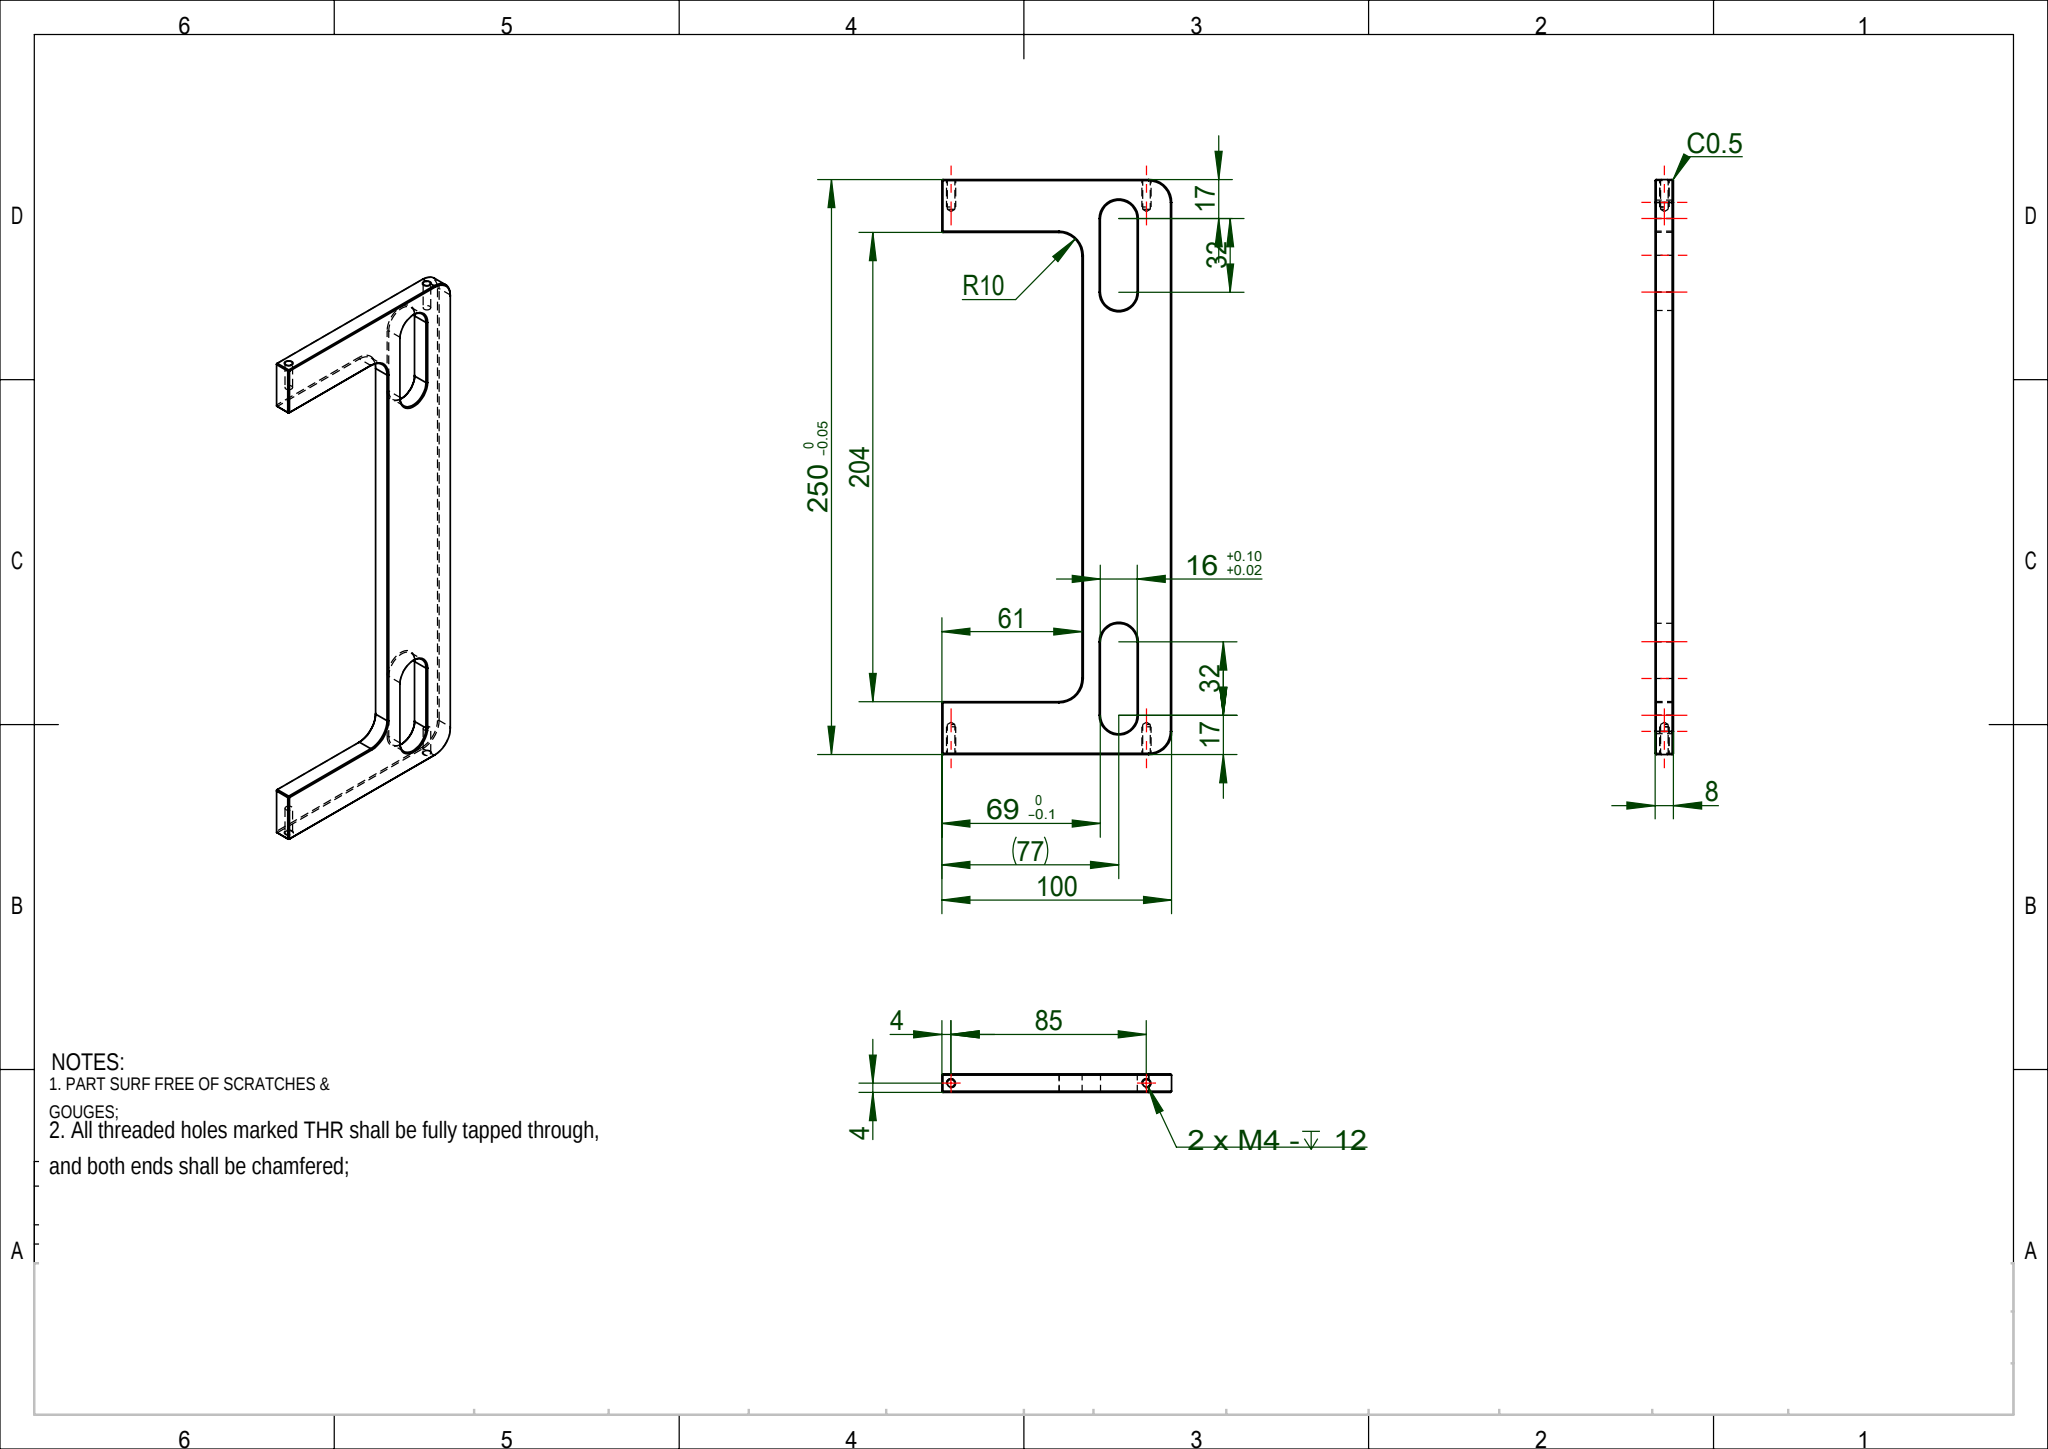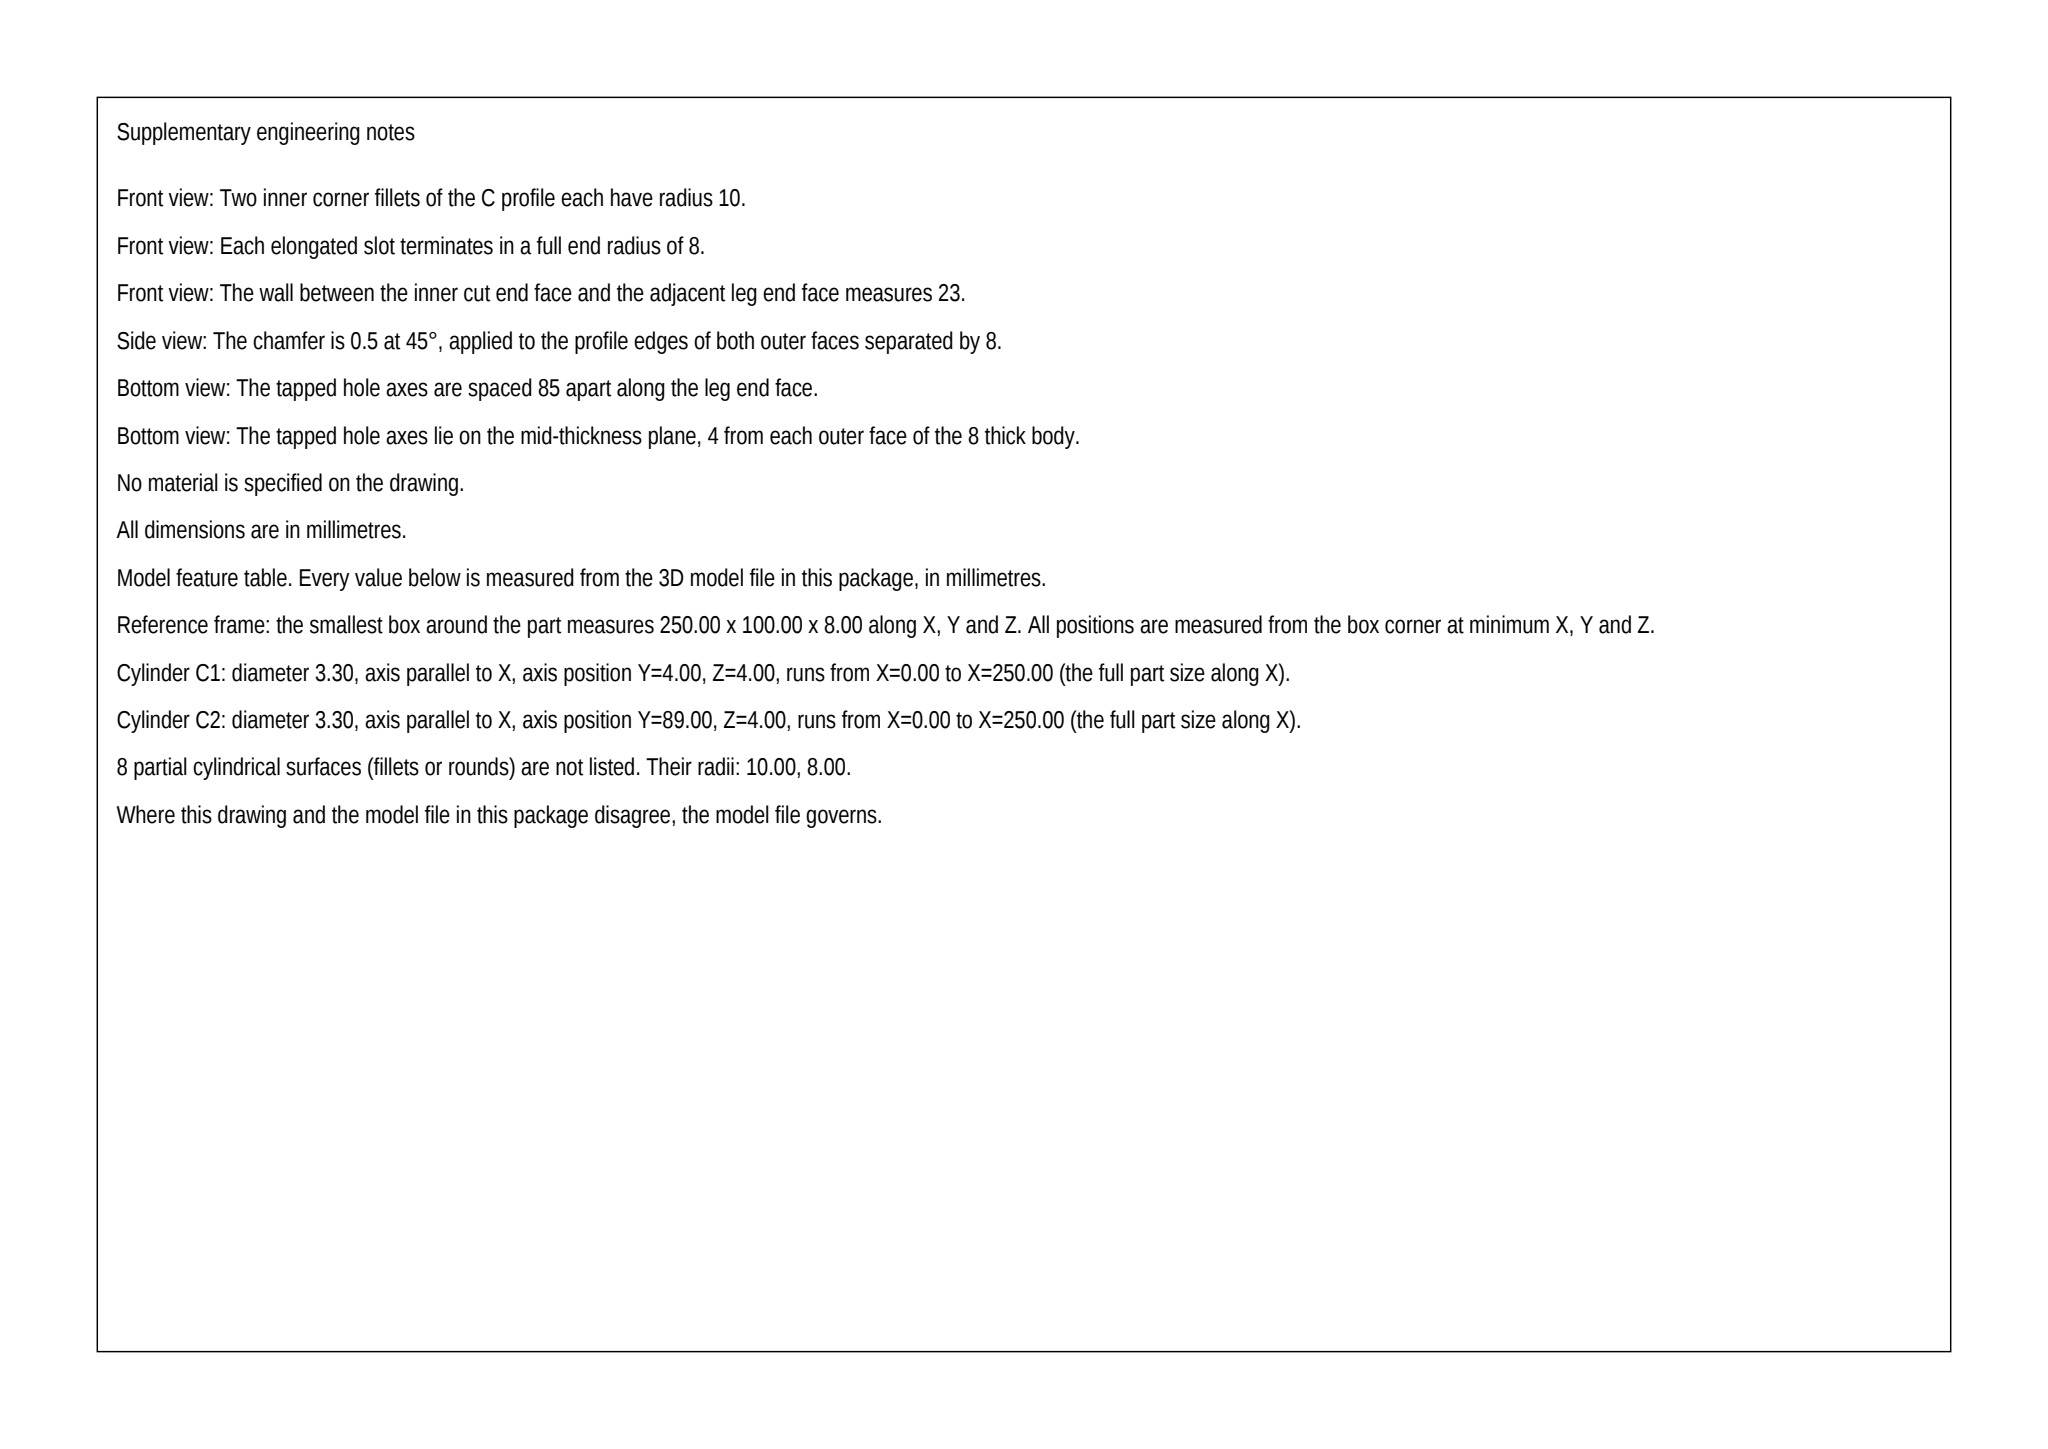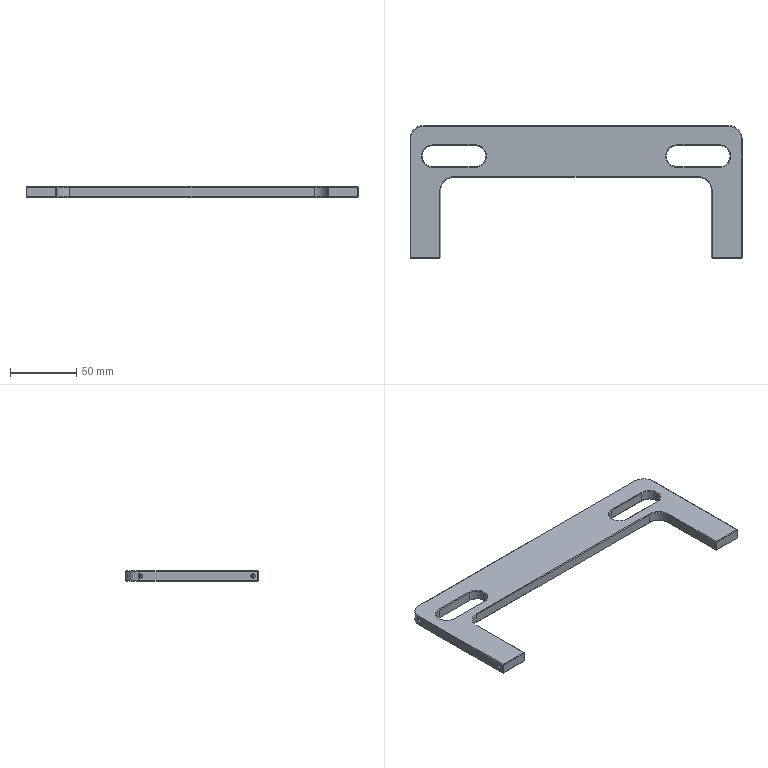Part | SolidWorks | mm | 1 solid | 96 faces | box 250 x 100 x 8 mm | volume 88321 mm3 | plane 50 | cone 28 | cylinder 18 | commonest cylinder face diameters 3.3 x8 16 x6 20 x4
Drawing notes:
INNER CORNER FILLETS: 2X R10 | from the solid: Inner profile corners at x=23 & x=227 meeting y=61 face are equal R10 fillets (2 places) in STEP solid
ARM THK 23 EA END; 204 NOTCH CTRD IN 250 (SYM) | from the solid: x-planes at 0, 23, 227, 250: ends 23 thk, inner span 204 centered
4X M4 TAPPED HOLE DP 12 (Ø3.3 DRILL DP 13), BOTH ENDS: TWO HOLES IN EACH 100 x 8 END FACE AT X=0 AND X=250; HOLE AXES PARALLEL TO 250 LENGTH, LOCATED 4 AND 89 FROM THE Y=0 EDGE (85 APART) AND 4 FROM THE Z=0 FACE (MID-THICKNESS). BOTH ENDS CHAMFERED. | from the solid: cylinders dia 3.3 axis x at [y=4,z=4] length 13 (count 4) and [y=89,z=4] length 13 (count 4); 118° cone ref dia 3.3 count 8; bbox 250 x 100 x 8; axis planes x=0 and x=250